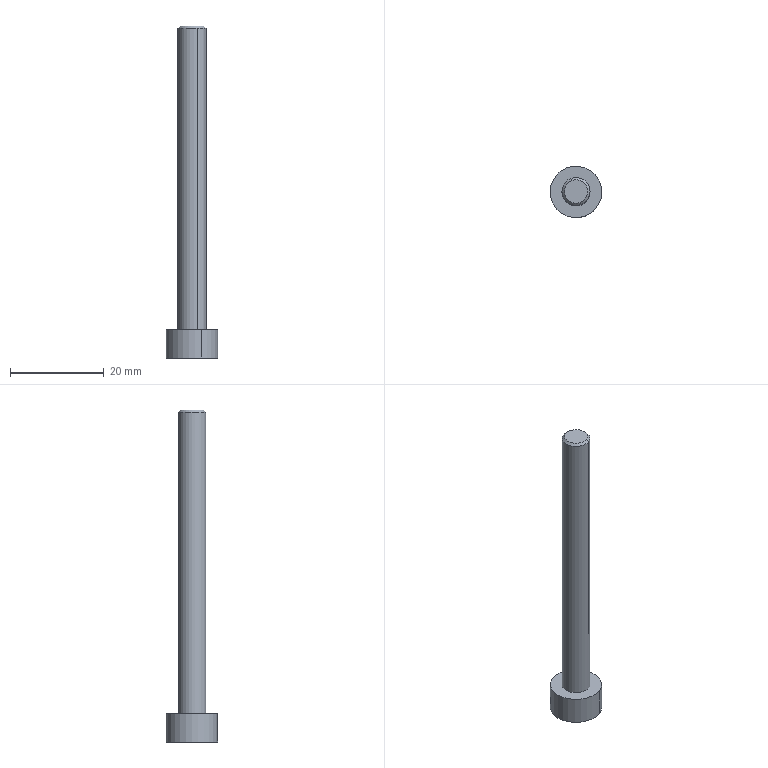Component | SolidWorks | ScrewM6X65-1 | 1 solid | 9 faces | box 11 x 11 x 71 mm | volume 2406 mm3 | cylinder 4 | plane 3 | cone 2 | commonest cylinder face diameters 6 x2 11 x2
build123d program:
from build123d import *

# Parameters (mm, degrees)
CHAMFER1_SIZE = 0.5


with BuildPart() as part:
    # Sketch1 → Revolve1 (revolve)
    with BuildSketch(Plane.XY, mode=Mode.PRIVATE) as revolve1_sk:
        Polygon((0, 0), (-5.5, 0), (-5.5, -6), (-3, -6), (-3, -71), (0, -71), align=None)
    revolve(revolve1_sk.sketch.rotate(Axis((0, 56.699, 0), (0, -1, 0)), 270), axis=Axis((0, 56.699, 0), (0, -1, 0)))

    # Chamfer1
    chamfer1_edges = [part.edges().sort_by_distance(p)[0] for p in [
        (0, -71, -3),
    ]]
    chamfer(chamfer1_edges, length=CHAMFER1_SIZE)


solid = part.part

# Placed as in the assembly
solid = solid.moved(Location((71.181, 6.396, -3), (-90, 0, 0)))
STEP:
#1=CARTESIAN_POINT('',(2.838,0.16,2.677));
#2=VERTEX_POINT('',#1);
#3=CARTESIAN_POINT('',(2.767,0.3436,2.677));
#4=VERTEX_POINT('',#3);
#5=CARTESIAN_POINT('',(2.802,0.2518,2.677));
#6=DIRECTION('',(0.,0.,1.));
#7=DIRECTION('',(0.3603,-0.9328,0.));
#8=AXIS2_PLACEMENT_3D('',#5,#6,#7);
#9=CIRCLE('',#8,0.09843);
#10=EDGE_CURVE('',#2,#4,#9,.T.);
#11=ORIENTED_EDGE('',*,*,#10,.F.);
#12=CARTESIAN_POINT('',(2.845,0.1416,2.657));
#13=VERTEX_POINT('',#12);
#14=CARTESIAN_POINT('',(2.845,0.1416,2.657));
#15=DIRECTION('',(0.2548,-0.6596,-0.7071));
#16=VECTOR('',#15,39.37);
#17=LINE('',#14,#16);
#18=EDGE_CURVE('',#2,#13,#17,.T.);
#19=ORIENTED_EDGE('',*,*,#18,.T.);
#20=CARTESIAN_POINT('',(2.76,0.362,2.657));
#21=VERTEX_POINT('',#20);
#22=CARTESIAN_POINT('',(2.802,0.2518,2.657));
#23=DIRECTION('',(0.,0.,-1.));
#24=DIRECTION('',(0.3603,-0.9328,0.));
#25=AXIS2_PLACEMENT_3D('',#22,#23,#24);
#26=CIRCLE('',#25,0.1181);
#27=EDGE_CURVE('',#21,#13,#26,.T.);
#28=ORIENTED_EDGE('',*,*,#27,.F.);
#29=CARTESIAN_POINT('',(2.76,0.362,2.657));
#30=DIRECTION('',(-0.2548,0.6596,-0.7071));
#31=VECTOR('',#30,39.37);
#32=LINE('',#29,#31);
#33=EDGE_CURVE('',#4,#21,#32,.T.);
#34=ORIENTED_EDGE('',*,*,#33,.F.);
#35=EDGE_LOOP('',(#11,#19,#28,#34));
#36=FACE_OUTER_BOUND('',#35,.T.);
#37=CARTESIAN_POINT('',(2.802,0.2518,2.657));
#38=DIRECTION('',(0.,0.,-1.));
#39=DIRECTION('',(-0.3603,0.9328,0.));
#40=AXIS2_PLACEMENT_3D('',#37,#38,#39);
#41=CONICAL_SURFACE('',#40,0.1181,0.7854);
#42=ADVANCED_FACE('',(#36),#41,.T.);
#43=ORIENTED_EDGE('',*,*,#27,.T.);
#44=CARTESIAN_POINT('',(2.845,0.1416,0.1181));
#45=VERTEX_POINT('',#44);
#46=CARTESIAN_POINT('',(2.845,0.1416,-2.35));
#47=DIRECTION('',(0.,0.,-1.));
#48=VECTOR('',#47,39.37);
#49=LINE('',#46,#48);
#50=EDGE_CURVE('',#13,#45,#49,.T.);
#51=ORIENTED_EDGE('',*,*,#50,.T.);
#52=CARTESIAN_POINT('',(2.76,0.362,0.1181));
#53=VERTEX_POINT('',#52);
#54=CARTESIAN_POINT('',(2.802,0.2518,0.1181));
#55=DIRECTION('',(0.,0.,-1.));
#56=DIRECTION('',(-0.3603,0.9328,0.));
#57=AXIS2_PLACEMENT_3D('',#54,#55,#56);
#58=CIRCLE('',#57,0.1181);
#59=EDGE_CURVE('',#53,#45,#58,.T.);
#60=ORIENTED_EDGE('',*,*,#59,.F.);
#61=CARTESIAN_POINT('',(2.76,0.362,-2.35));
#62=DIRECTION('',(0.,0.,-1.));
#63=VECTOR('',#62,39.37);
#64=LINE('',#61,#63);
#65=EDGE_CURVE('',#21,#53,#64,.T.);
#66=ORIENTED_EDGE('',*,*,#65,.F.);
#67=EDGE_LOOP('',(#43,#51,#60,#66));
#68=FACE_OUTER_BOUND('',#67,.T.);
#69=CARTESIAN_POINT('',(2.802,0.2518,-2.35));
#70=DIRECTION('',(0.,0.,-1.));
#71=DIRECTION('',(-0.3603,0.9328,0.));
#72=AXIS2_PLACEMENT_3D('',#69,#70,#71);
#73=CYLINDRICAL_SURFACE('',#72,0.1181);
#74=ADVANCED_FACE('',(#68),#73,.T.);
#75=CARTESIAN_POINT('',(2.724,0.4538,0.1181));
#76=VERTEX_POINT('',#75);
#77=CARTESIAN_POINT('',(2.88,0.04981,0.1181));
#78=VERTEX_POINT('',#77);
#79=CARTESIAN_POINT('',(2.802,0.2518,0.1181));
#80=DIRECTION('',(0.,0.,-1.));
#81=DIRECTION('',(-0.3603,0.9328,0.));
#82=AXIS2_PLACEMENT_3D('',#79,#80,#81);
#83=CIRCLE('',#82,0.2165);
#84=EDGE_CURVE('',#76,#78,#83,.T.);
#85=ORIENTED_EDGE('',*,*,#84,.T.);
#86=CARTESIAN_POINT('',(2.88,0.04981,-0.1181));
#87=VERTEX_POINT('',#86);
#88=CARTESIAN_POINT('',(2.88,0.04981,-2.35));
#89=DIRECTION('',(0.,0.,-1.));
#90=VECTOR('',#89,39.37);
#91=LINE('',#88,#90);
#92=EDGE_CURVE('',#78,#87,#91,.T.);
#93=ORIENTED_EDGE('',*,*,#92,.T.);
#94=CARTESIAN_POINT('',(2.724,0.4538,-0.1181));
#95=VERTEX_POINT('',#94);
#96=CARTESIAN_POINT('',(2.802,0.2518,-0.1181));
#97=DIRECTION('',(0.,0.,-1.));
#98=DIRECTION('',(-0.3603,0.9328,0.));
#99=AXIS2_PLACEMENT_3D('',#96,#97,#98);
#100=CIRCLE('',#99,0.2165);
#101=EDGE_CURVE('',#95,#87,#100,.T.);
#102=ORIENTED_EDGE('',*,*,#101,.F.);
#103=CARTESIAN_POINT('',(2.724,0.4538,-2.35));
#104=DIRECTION('',(0.,0.,-1.));
#105=VECTOR('',#104,39.37);
#106=LINE('',#103,#105);
#107=EDGE_CURVE('',#76,#95,#106,.T.);
#108=ORIENTED_EDGE('',*,*,#107,.F.);
#109=EDGE_LOOP('',(#85,#93,#102,#108));
#110=FACE_OUTER_BOUND('',#109,.T.);
#111=CARTESIAN_POINT('',(2.802,0.2518,-2.35));
#112=DIRECTION('',(0.,0.,-1.));
#113=DIRECTION('',(-0.3603,0.9328,0.));
#114=AXIS2_PLACEMENT_3D('',#111,#112,#113);
#115=CYLINDRICAL_SURFACE('',#114,0.2165);
#116=ADVANCED_FACE('',(#110),#115,.T.);
#117=ORIENTED_EDGE('',*,*,#101,.T.);
#118=CARTESIAN_POINT('',(2.802,0.2518,-0.1181));
#119=DIRECTION('',(0.,0.,-1.));
#120=DIRECTION('',(-0.3603,0.9328,0.));
#121=AXIS2_PLACEMENT_3D('',#118,#119,#120);
#122=CIRCLE('',#121,0.2165);
#123=EDGE_CURVE('',#87,#95,#122,.T.);
#124=ORIENTED_EDGE('',*,*,#123,.T.);
#125=EDGE_LOOP('',(#117,#124));
#126=FACE_OUTER_BOUND('',#125,.T.);
#127=CARTESIAN_POINT('',(2.802,0.2518,-0.1181));
#128=DIRECTION('',(0.,0.,-1.));
#129=DIRECTION('',(-0.3603,0.9328,0.));
#130=AXIS2_PLACEMENT_3D('',#127,#128,#129);
#131=PLANE('',#130);
#132=ADVANCED_FACE('',(#126),#131,.T.);
#133=ORIENTED_EDGE('',*,*,#92,.F.);
#134=CARTESIAN_POINT('',(2.802,0.2518,0.1181));
#135=DIRECTION('',(0.,0.,-1.));
#136=DIRECTION('',(-0.3603,0.9328,0.));
#137=AXIS2_PLACEMENT_3D('',#134,#135,#136);
#138=CIRCLE('',#137,0.2165);
#139=EDGE_CURVE('',#78,#76,#138,.T.);
#140=ORIENTED_EDGE('',*,*,#139,.T.);
#141=ORIENTED_EDGE('',*,*,#107,.T.);
#142=ORIENTED_EDGE('',*,*,#123,.F.);
#143=EDGE_LOOP('',(#133,#140,#141,#142));
#144=FACE_OUTER_BOUND('',#143,.T.);
#145=CARTESIAN_POINT('',(2.802,0.2518,-2.35));
#146=DIRECTION('',(0.,0.,-1.));
#147=DIRECTION('',(-0.3603,0.9328,0.));
#148=AXIS2_PLACEMENT_3D('',#145,#146,#147);
#149=CYLINDRICAL_SURFACE('',#148,0.2165);
#150=ADVANCED_FACE('',(#144),#149,.T.);
#151=ORIENTED_EDGE('',*,*,#59,.T.);
#152=CARTESIAN_POINT('',(2.802,0.2518,0.1181));
#153=DIRECTION('',(0.,0.,-1.));
#154=DIRECTION('',(-0.3603,0.9328,0.));
#155=AXIS2_PLACEMENT_3D('',#152,#153,#154);
#156=CIRCLE('',#155,0.1181);
#157=EDGE_CURVE('',#45,#53,#156,.T.);
#158=ORIENTED_EDGE('',*,*,#157,.T.);
#159=EDGE_LOOP('',(#151,#158));
#160=FACE_BOUND('',#159,.T.);
#161=ORIENTED_EDGE('',*,*,#84,.F.);
#162=ORIENTED_EDGE('',*,*,#139,.F.);
#163=EDGE_LOOP('',(#161,#162));
#164=FACE_OUTER_BOUND('',#163,.T.);
#165=CARTESIAN_POINT('',(2.6,0.1738,0.1181));
#166=DIRECTION('',(0.,0.,1.));
#167=DIRECTION('',(0.3603,-0.9328,0.));
#168=AXIS2_PLACEMENT_3D('',#165,#166,#167);
#169=PLANE('',#168);
#170=ADVANCED_FACE('',(#160,#164),#169,.T.);
#171=ORIENTED_EDGE('',*,*,#50,.F.);
#172=CARTESIAN_POINT('',(2.802,0.2518,2.657));
#173=DIRECTION('',(0.,0.,-1.));
#174=DIRECTION('',(0.3603,-0.9328,0.));
#175=AXIS2_PLACEMENT_3D('',#172,#173,#174);
#176=CIRCLE('',#175,0.1181);
#177=EDGE_CURVE('',#13,#21,#176,.T.);
#178=ORIENTED_EDGE('',*,*,#177,.T.);
#179=ORIENTED_EDGE('',*,*,#65,.T.);
#180=ORIENTED_EDGE('',*,*,#157,.F.);
#181=EDGE_LOOP('',(#171,#178,#179,#180));
#182=FACE_OUTER_BOUND('',#181,.T.);
#183=CARTESIAN_POINT('',(2.802,0.2518,-2.35));
#184=DIRECTION('',(0.,0.,-1.));
#185=DIRECTION('',(-0.3603,0.9328,0.));
#186=AXIS2_PLACEMENT_3D('',#183,#184,#185);
#187=CYLINDRICAL_SURFACE('',#186,0.1181);
#188=ADVANCED_FACE('',(#182),#187,.T.);
#189=CARTESIAN_POINT('',(2.802,0.2518,2.677));
#190=DIRECTION('',(0.,0.,1.));
#191=DIRECTION('',(0.3603,-0.9328,0.));
#192=AXIS2_PLACEMENT_3D('',#189,#190,#191);
#193=CIRCLE('',#192,0.09843);
#194=EDGE_CURVE('',#4,#2,#193,.T.);
#195=ORIENTED_EDGE('',*,*,#194,.T.);
#196=ORIENTED_EDGE('',*,*,#10,.T.);
#197=EDGE_LOOP('',(#195,#196));
#198=FACE_OUTER_BOUND('',#197,.T.);
#199=CARTESIAN_POINT('',(2.692,0.2092,2.677));
#200=DIRECTION('',(0.,0.,1.));
#201=DIRECTION('',(0.3603,-0.9328,0.));
#202=AXIS2_PLACEMENT_3D('',#199,#200,#201);
#203=PLANE('',#202);
#204=ADVANCED_FACE('',(#198),#203,.T.);
#205=ORIENTED_EDGE('',*,*,#18,.F.);
#206=ORIENTED_EDGE('',*,*,#194,.F.);
#207=ORIENTED_EDGE('',*,*,#33,.T.);
#208=ORIENTED_EDGE('',*,*,#177,.F.);
#209=EDGE_LOOP('',(#205,#206,#207,#208));
#210=FACE_OUTER_BOUND('',#209,.T.);
#211=CARTESIAN_POINT('',(2.802,0.2518,2.657));
#212=DIRECTION('',(0.,0.,-1.));
#213=DIRECTION('',(-0.3603,0.9328,0.));
#214=AXIS2_PLACEMENT_3D('',#211,#212,#213);
#215=CONICAL_SURFACE('',#214,0.1181,0.7854);
#216=ADVANCED_FACE('',(#210),#215,.T.);
#217=CLOSED_SHELL('',(#42,#74,#116,#132,#150,#170,#188,#204,#216));
#218=MANIFOLD_SOLID_BREP('',#217);
#219=CARTESIAN_POINT('',(0.,0.,0.));
#220=DIRECTION('',(0.,0.,1.));
#221=DIRECTION('',(1.,0.,0.));
#222=AXIS2_PLACEMENT_3D('',#219,#220,#221);
#223=(LENGTH_UNIT()NAMED_UNIT(*)SI_UNIT($,.METRE.));
#224=LENGTH_MEASURE_WITH_UNIT(LENGTH_MEASURE(0.0254),#223);
#225=DIMENSIONAL_EXPONENTS(1.,0.,0.,0.,0.,0.,0.);
#226=(CONVERSION_BASED_UNIT('',#224)LENGTH_UNIT()NAMED_UNIT(#225));
#227=UNCERTAINTY_MEASURE_WITH_UNIT(LENGTH_MEASURE(0.00001),#226,'','');
#228=(NAMED_UNIT(*)PLANE_ANGLE_UNIT()SI_UNIT($,.RADIAN.));
#229=(NAMED_UNIT(*)SI_UNIT($,.STERADIAN.)SOLID_ANGLE_UNIT());
#230=(GEOMETRIC_REPRESENTATION_CONTEXT(3)GLOBAL_UNCERTAINTY_ASSIGNED_CONTEXT((#227))GLOBAL_UNIT_ASSIGNED_CONTEXT((#226,#228,#229))REPRESENTATION_CONTEXT('',''));
#231=ADVANCED_BREP_SHAPE_REPRESENTATION('',(#218,#222),#230);
#232=COLOUR_RGB('',0.7922,0.8196,0.9333);
#233=FILL_AREA_STYLE_COLOUR('',#232);
#234=FILL_AREA_STYLE('',(#233));
#235=SURFACE_STYLE_FILL_AREA(#234);
#236=SURFACE_SIDE_STYLE('',(#235));
#237=SURFACE_STYLE_USAGE(.BOTH.,#236);
#238=PRESENTATION_STYLE_ASSIGNMENT((#237));
#239=STYLED_ITEM('',(#238),#218);
#240=(LENGTH_UNIT()NAMED_UNIT(*)SI_UNIT($,.METRE.));
#241=LENGTH_MEASURE_WITH_UNIT(LENGTH_MEASURE(0.0254),#240);
#242=DIMENSIONAL_EXPONENTS(1.,0.,0.,0.,0.,0.,0.);
#243=(CONVERSION_BASED_UNIT('',#241)LENGTH_UNIT()NAMED_UNIT(#242));
#244=UNCERTAINTY_MEASURE_WITH_UNIT(LENGTH_MEASURE(0.00001),#243,'','');
#245=(NAMED_UNIT(*)PLANE_ANGLE_UNIT()SI_UNIT($,.RADIAN.));
#246=(NAMED_UNIT(*)SI_UNIT($,.STERADIAN.)SOLID_ANGLE_UNIT());
#247=(GEOMETRIC_REPRESENTATION_CONTEXT(3)GLOBAL_UNCERTAINTY_ASSIGNED_CONTEXT((#244))GLOBAL_UNIT_ASSIGNED_CONTEXT((#243,#245,#246))REPRESENTATION_CONTEXT('',''));
#248=MECHANICAL_DESIGN_GEOMETRIC_PRESENTATION_REPRESENTATION('',(#239),#247);
#249=PRESENTATION_LAYER_ASSIGNMENT('','',(#239));